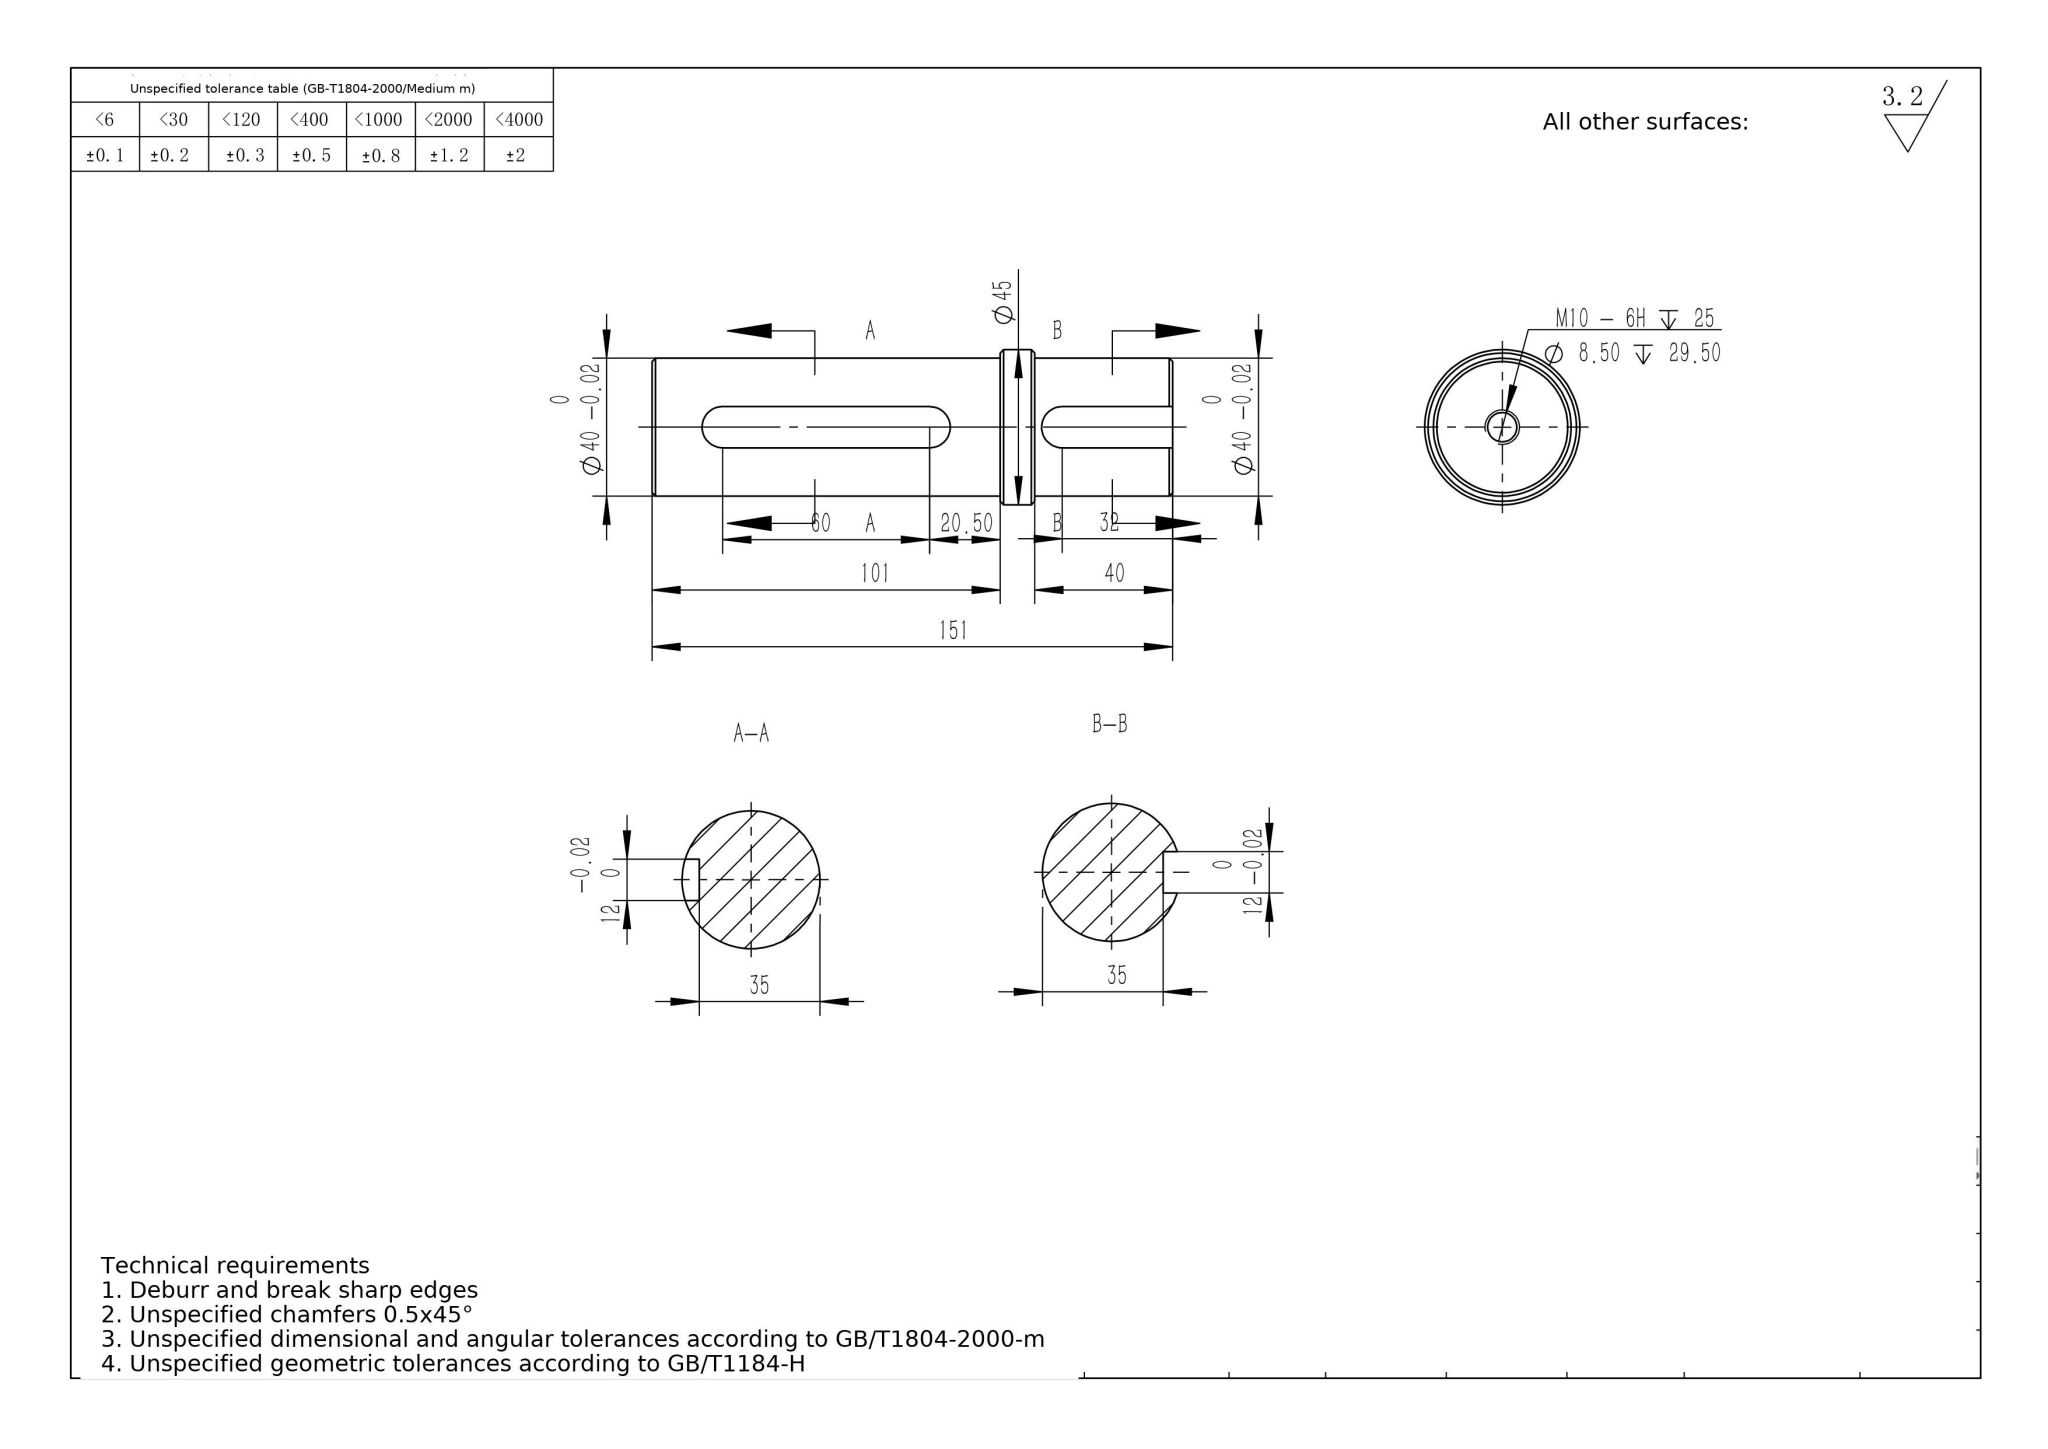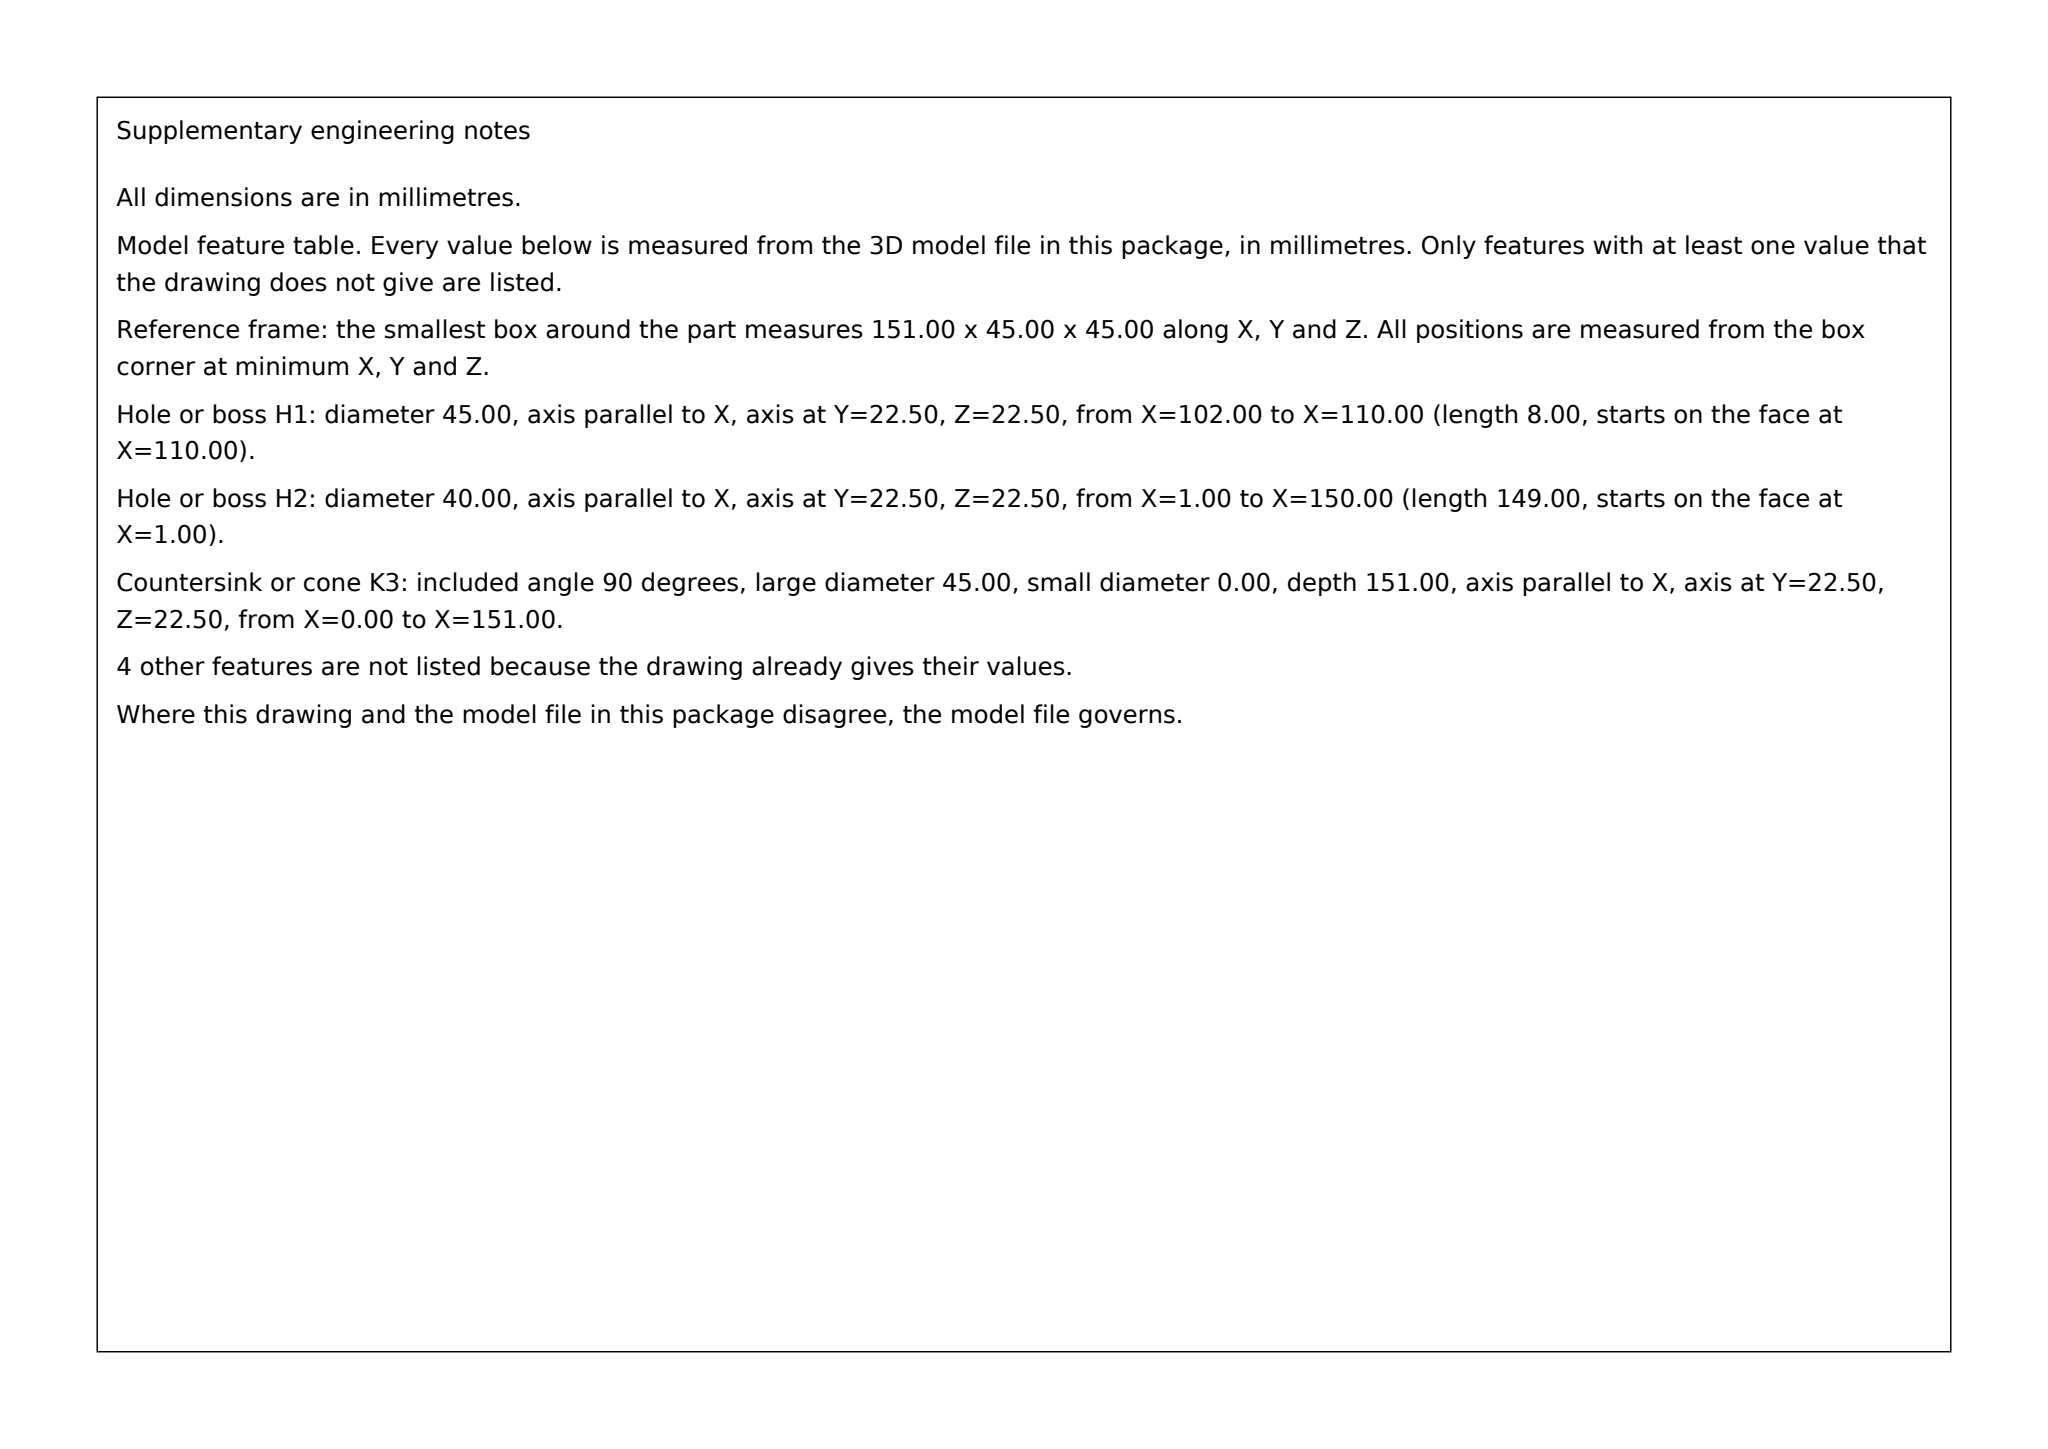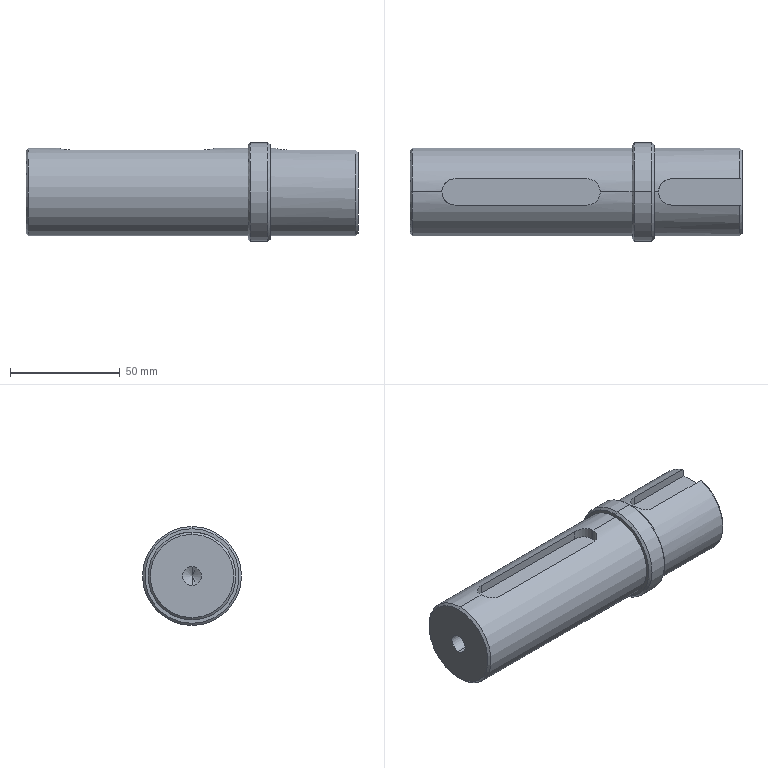Part | SolidWorks | mm | 1 solid | 31 faces | box 151 x 45 x 45 mm | volume 185117 mm3 | cylinder 12 | plane 10 | cone 9 | commonest cylinder face diameters 12 x4 40 x4 8.5 x2 45 x2
build123d program:
from build123d import *

# Parameters (mm, degrees)
M10_TAPPED_HOLE1_D     = 8.5
M10_TAPPED_HOLE1_DEPTH = 29.5
M10_TAPPED_HOLE1_TIP   = 2.554
CHAMFER1_SIZE          = 1
CUT_EXTRUDE1_START     = 20
CUT_EXTRUDE1_DEPTH     = 5


with BuildPart() as part:
    # Sketch1 → Revolve1 (revolve)
    with BuildSketch(Plane.XY, mode=Mode.PRIVATE) as revolve1_sk:
        Polygon((0, 0), (0, 20), (101, 20), (101, 22.5), (111, 22.5), (111, 20), (151, 20), (151, 0), align=None)
    revolve(revolve1_sk.sketch.rotate(Axis((0, 0, 0), (1, 0, 0)), 90), axis=Axis((0, 0, 0), (1, 0, 0)))

    # M10 Tapped Hole1
    with Locations(Plane.ZY):
        with Locations((0, 0)):
            Hole(M10_TAPPED_HOLE1_D / 2, depth=M10_TAPPED_HOLE1_DEPTH)
            with Locations((0, 0, -(M10_TAPPED_HOLE1_DEPTH + M10_TAPPED_HOLE1_TIP / 2))):  # 118° drill point
                Cone(0, M10_TAPPED_HOLE1_D / 2, M10_TAPPED_HOLE1_TIP, mode=Mode.SUBTRACT)

    # Chamfer1
    chamfer1_edges = [part.edges().sort_by_distance(p)[0] for p in [
        (151, 0, -20),
        (111, 0, -22.5),
        (101, 0, -22.5),
        (0, 0, -20),
    ]]
    chamfer(chamfer1_edges, length=CHAMFER1_SIZE)

    # Sketch4 → Cut-Extrude1 (cut)
    with BuildSketch(Plane.XY.offset(CUT_EXTRUDE1_START)):
        with BuildLine():
            Line((151, -6), (119, -6))
            ThreePointArc((119, -6), (113, 0), (119, 6))
            Line((119, 6), (151, 6))
            ThreePointArc((151, 6), (157, 0), (151, -6))
        make_face()
        with BuildLine():
            Line((20.5, 6), (80.5, 6))
            ThreePointArc((80.5, 6), (86.5, 0), (80.5, -6))
            Line((80.5, -6), (20.5, -6))
            ThreePointArc((20.5, -6), (14.5, 0), (20.5, 6))
        make_face()
    extrude(amount=-CUT_EXTRUDE1_DEPTH, mode=Mode.SUBTRACT)


solid = part.part